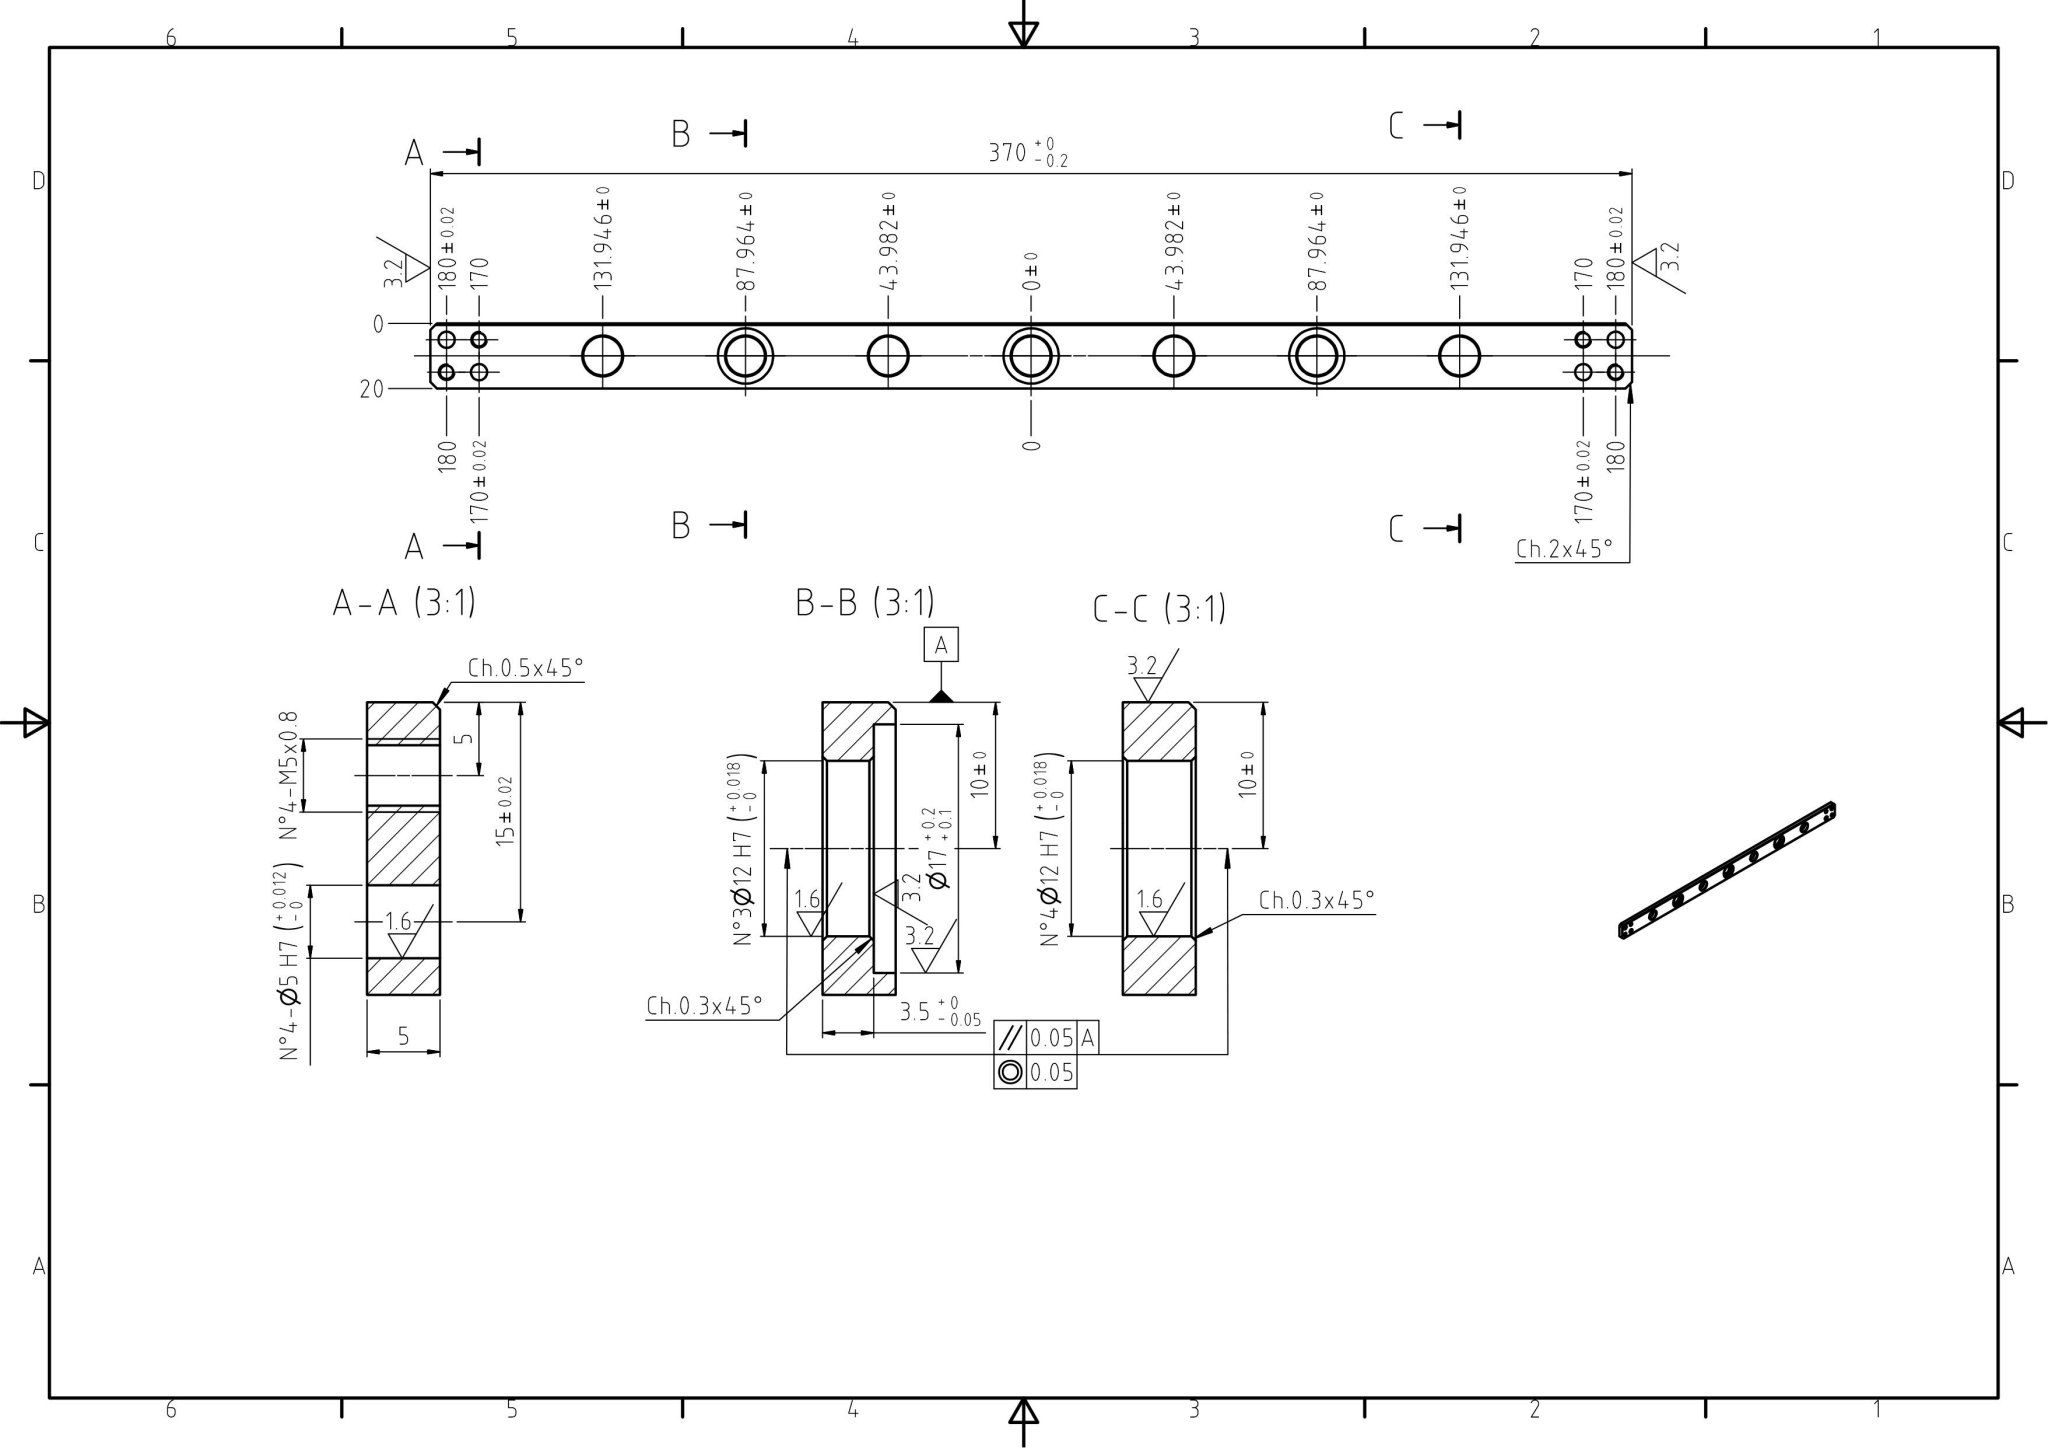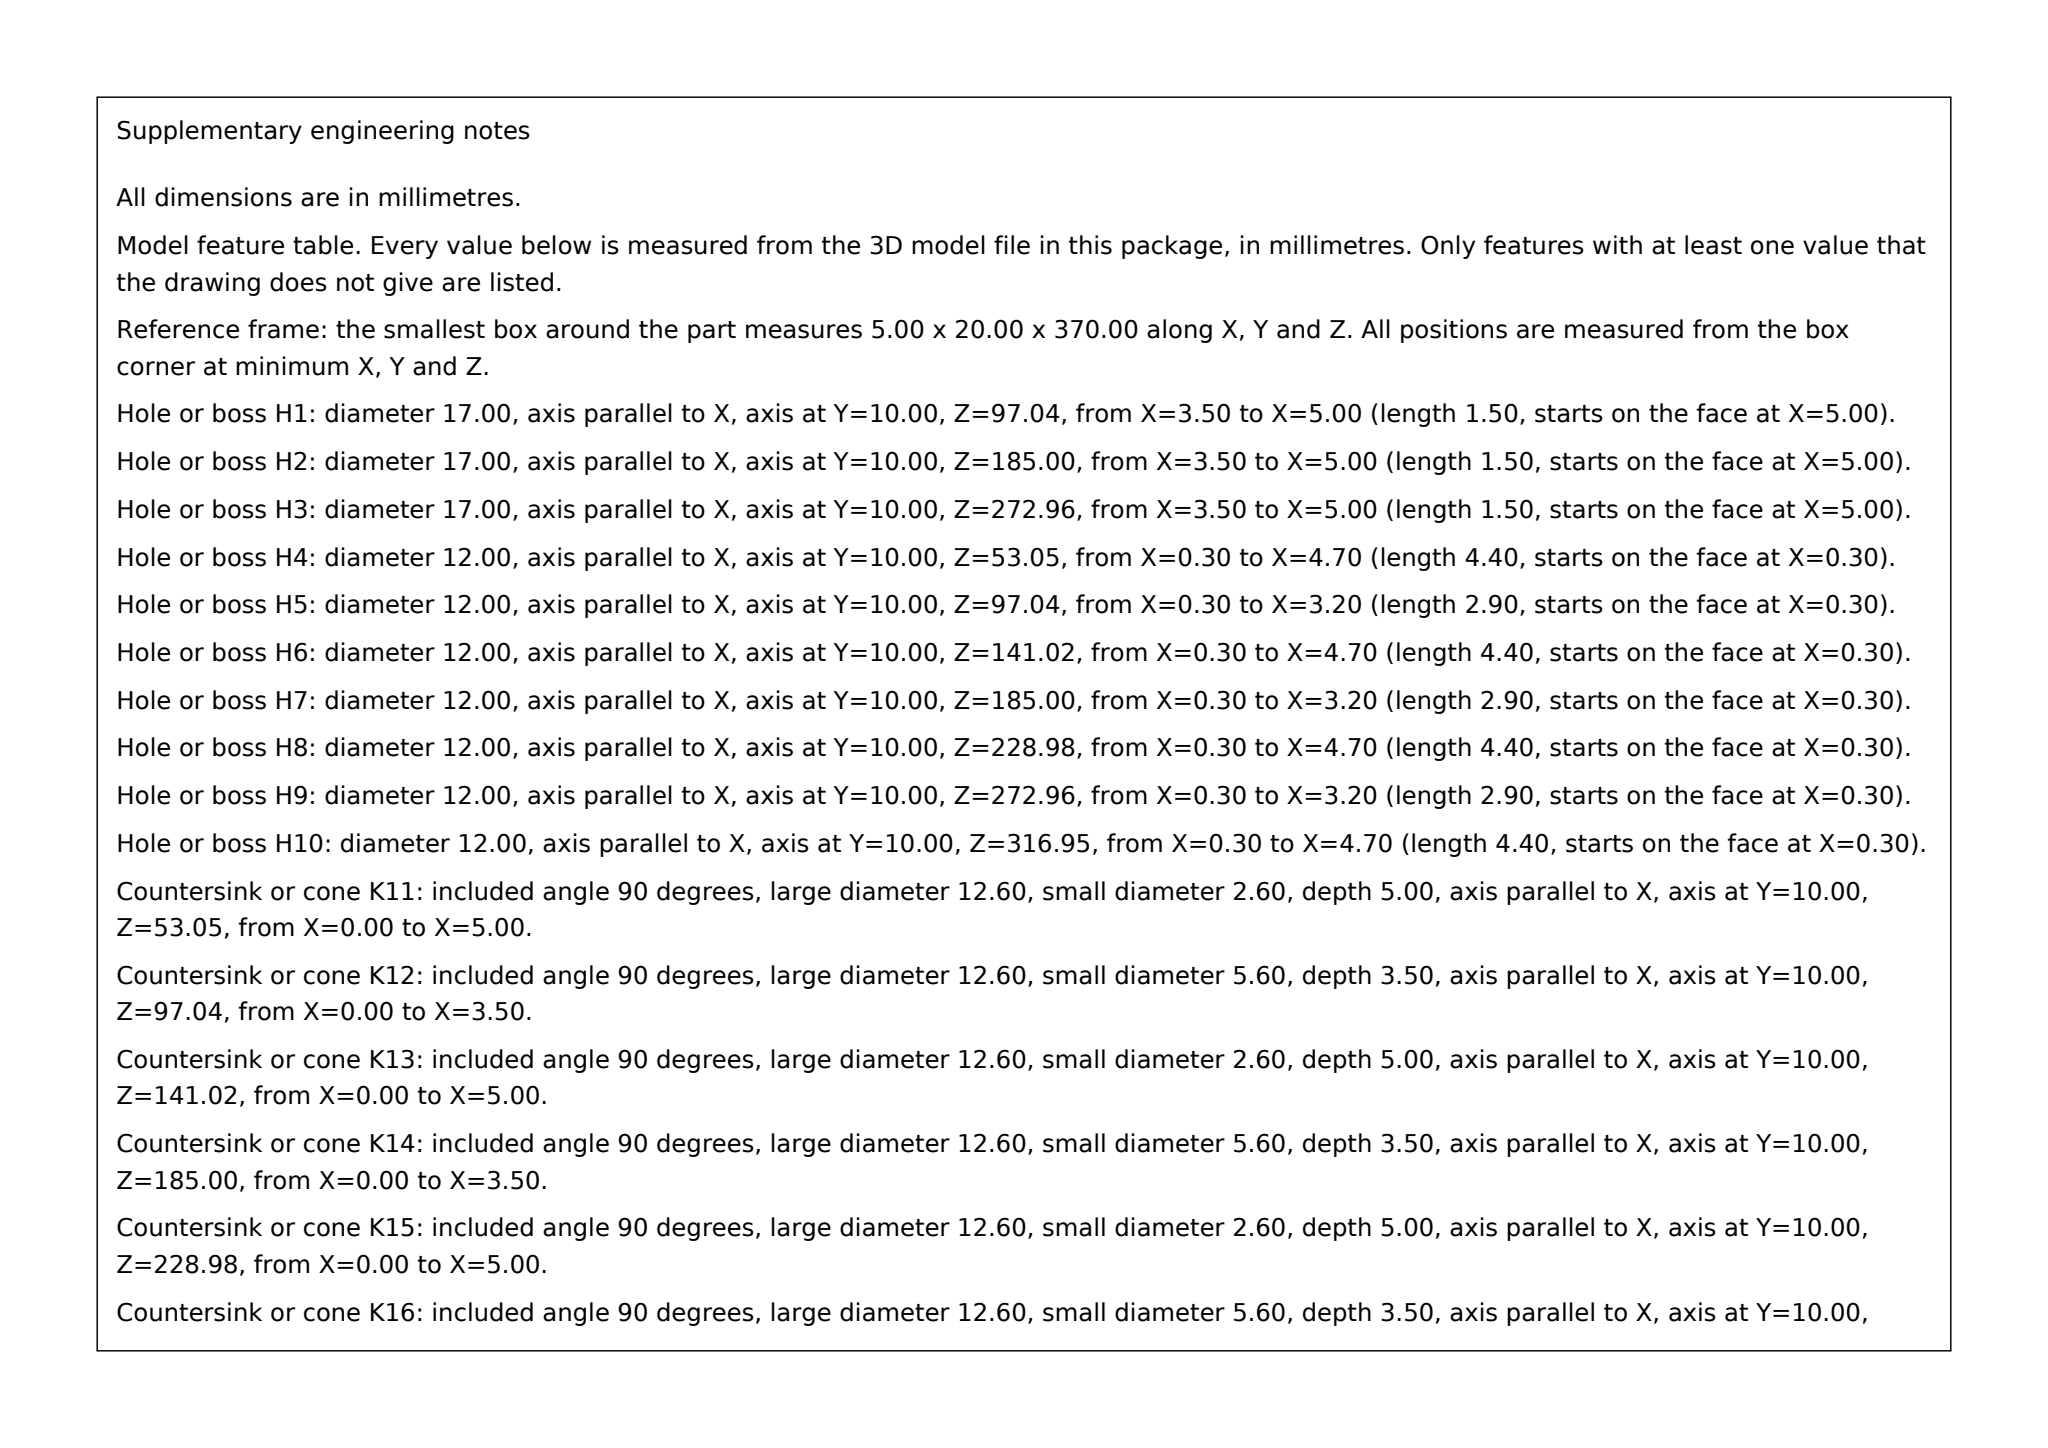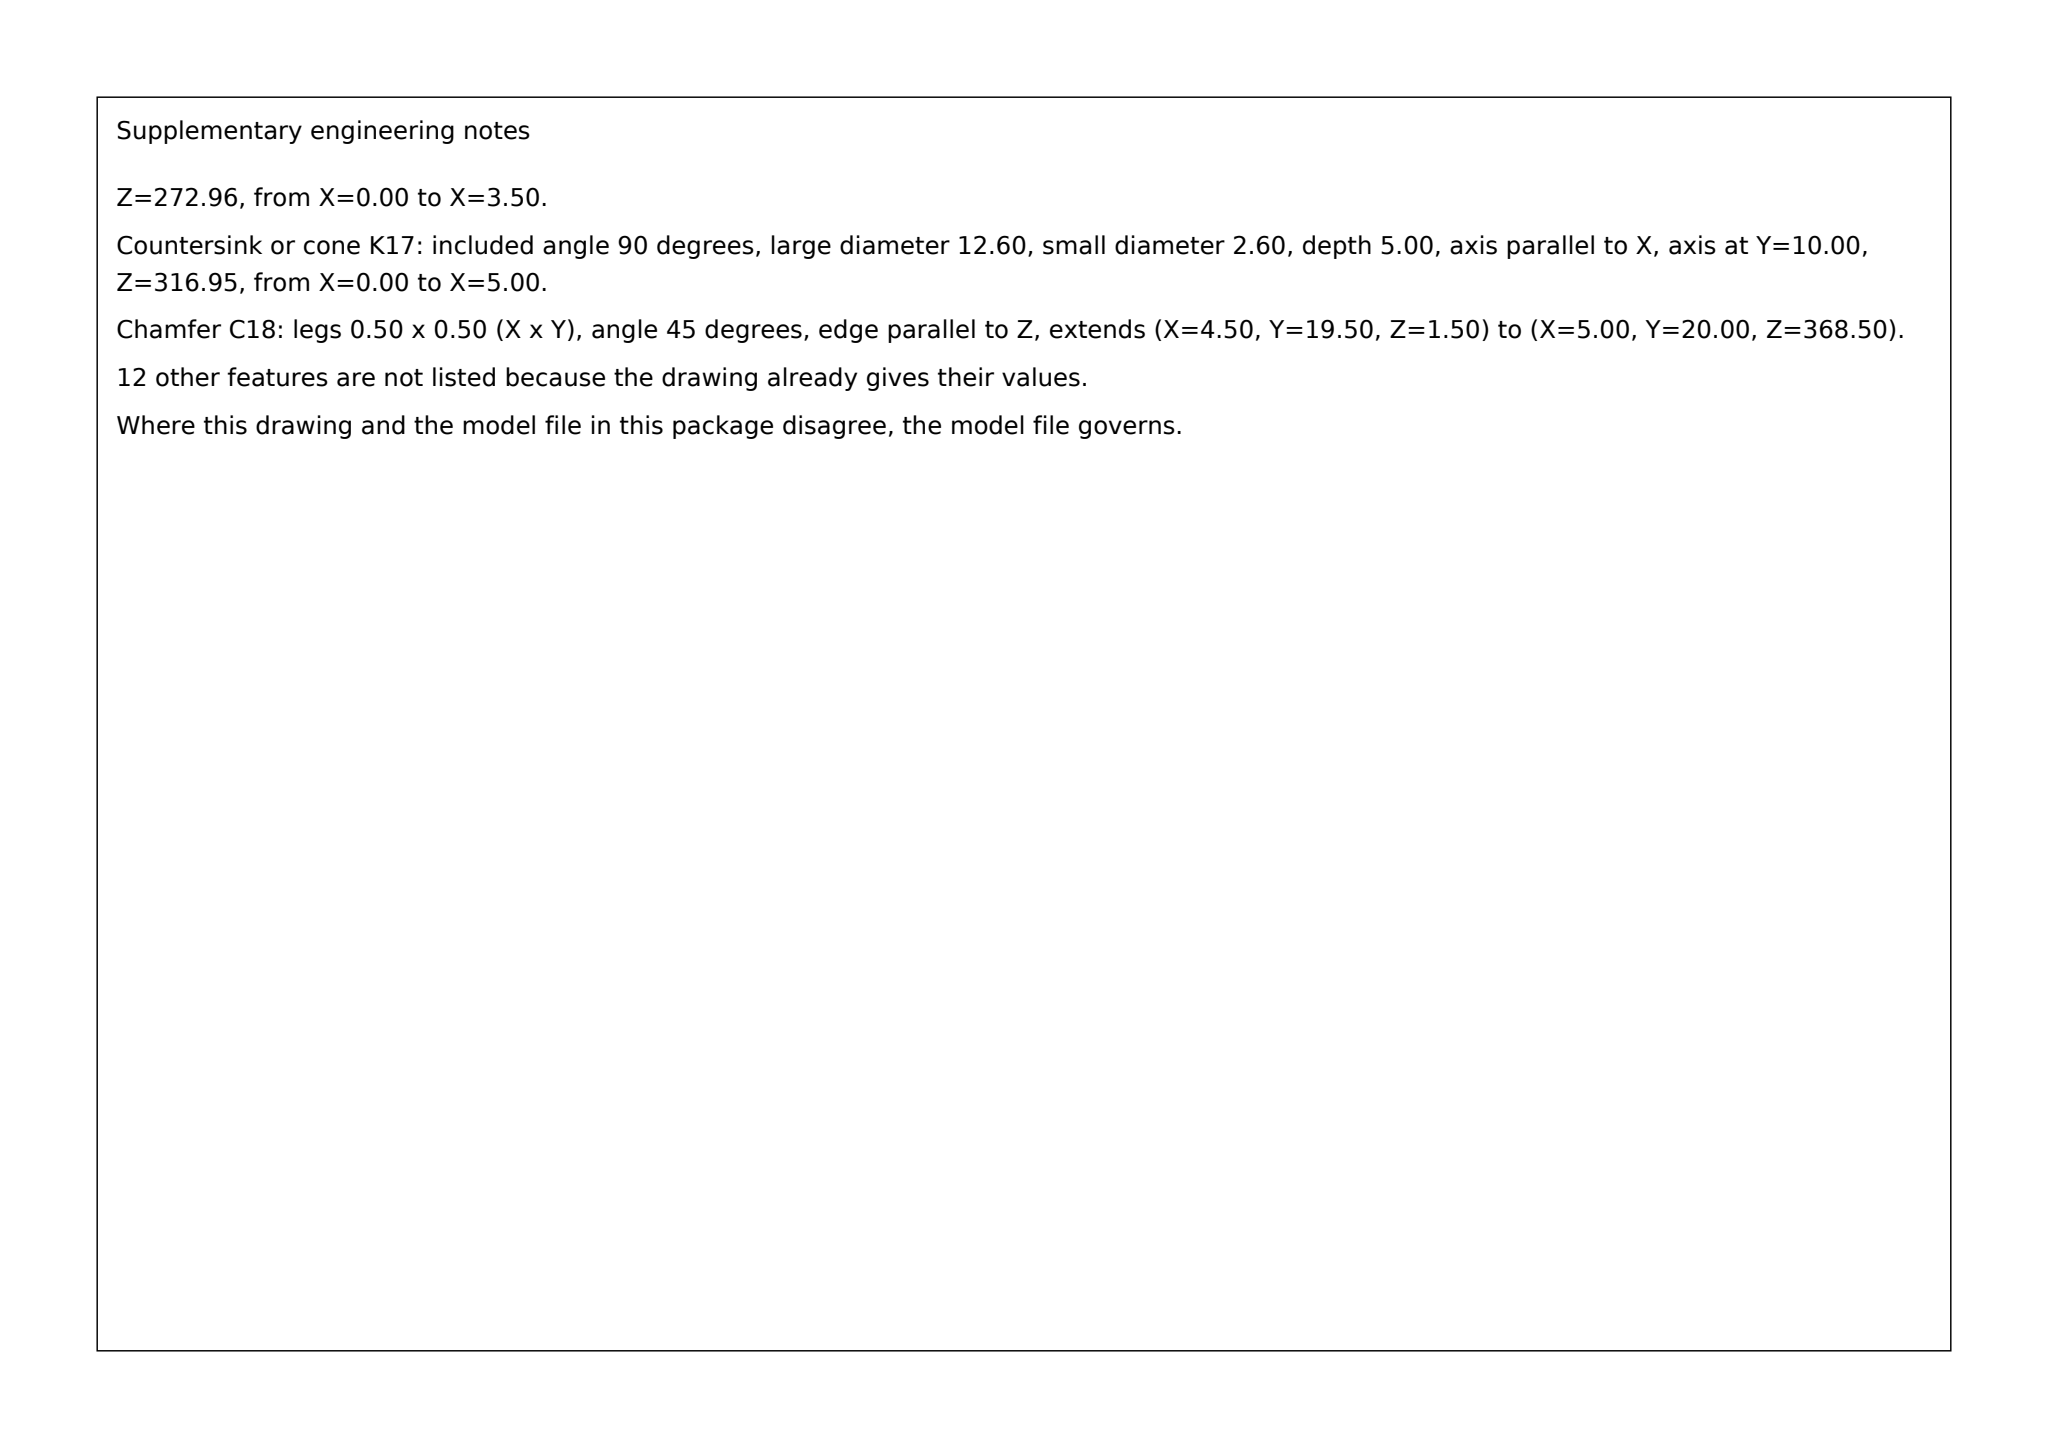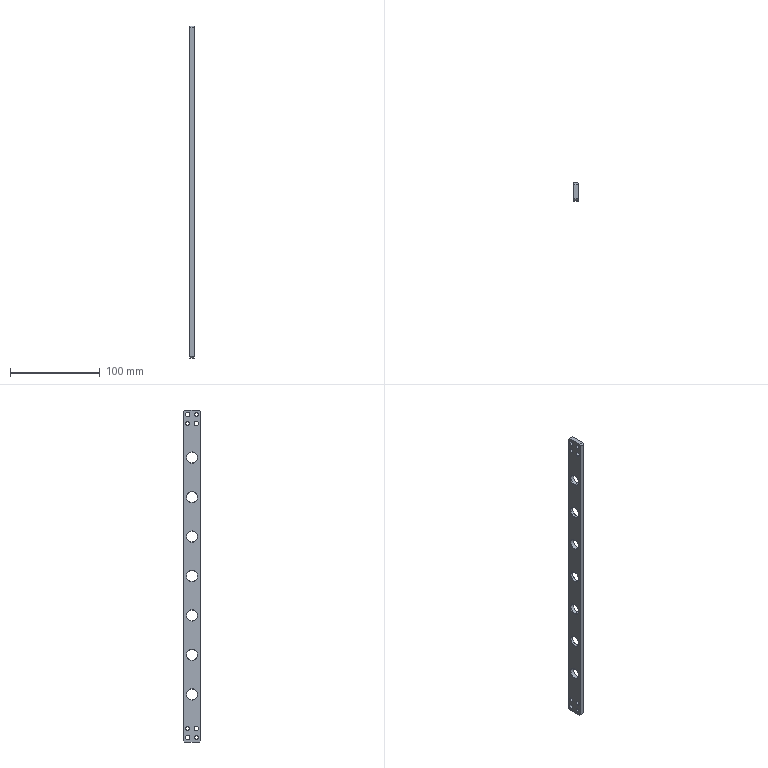Part | SolidWorks | mm | 1 solid | 78 faces | box 5 x 20 x 370 mm | volume 31758 mm3 | cylinder 36 | cone 28 | plane 14 | commonest cylinder face diameters 12 x14 5 x8 4.134 x8 17 x6